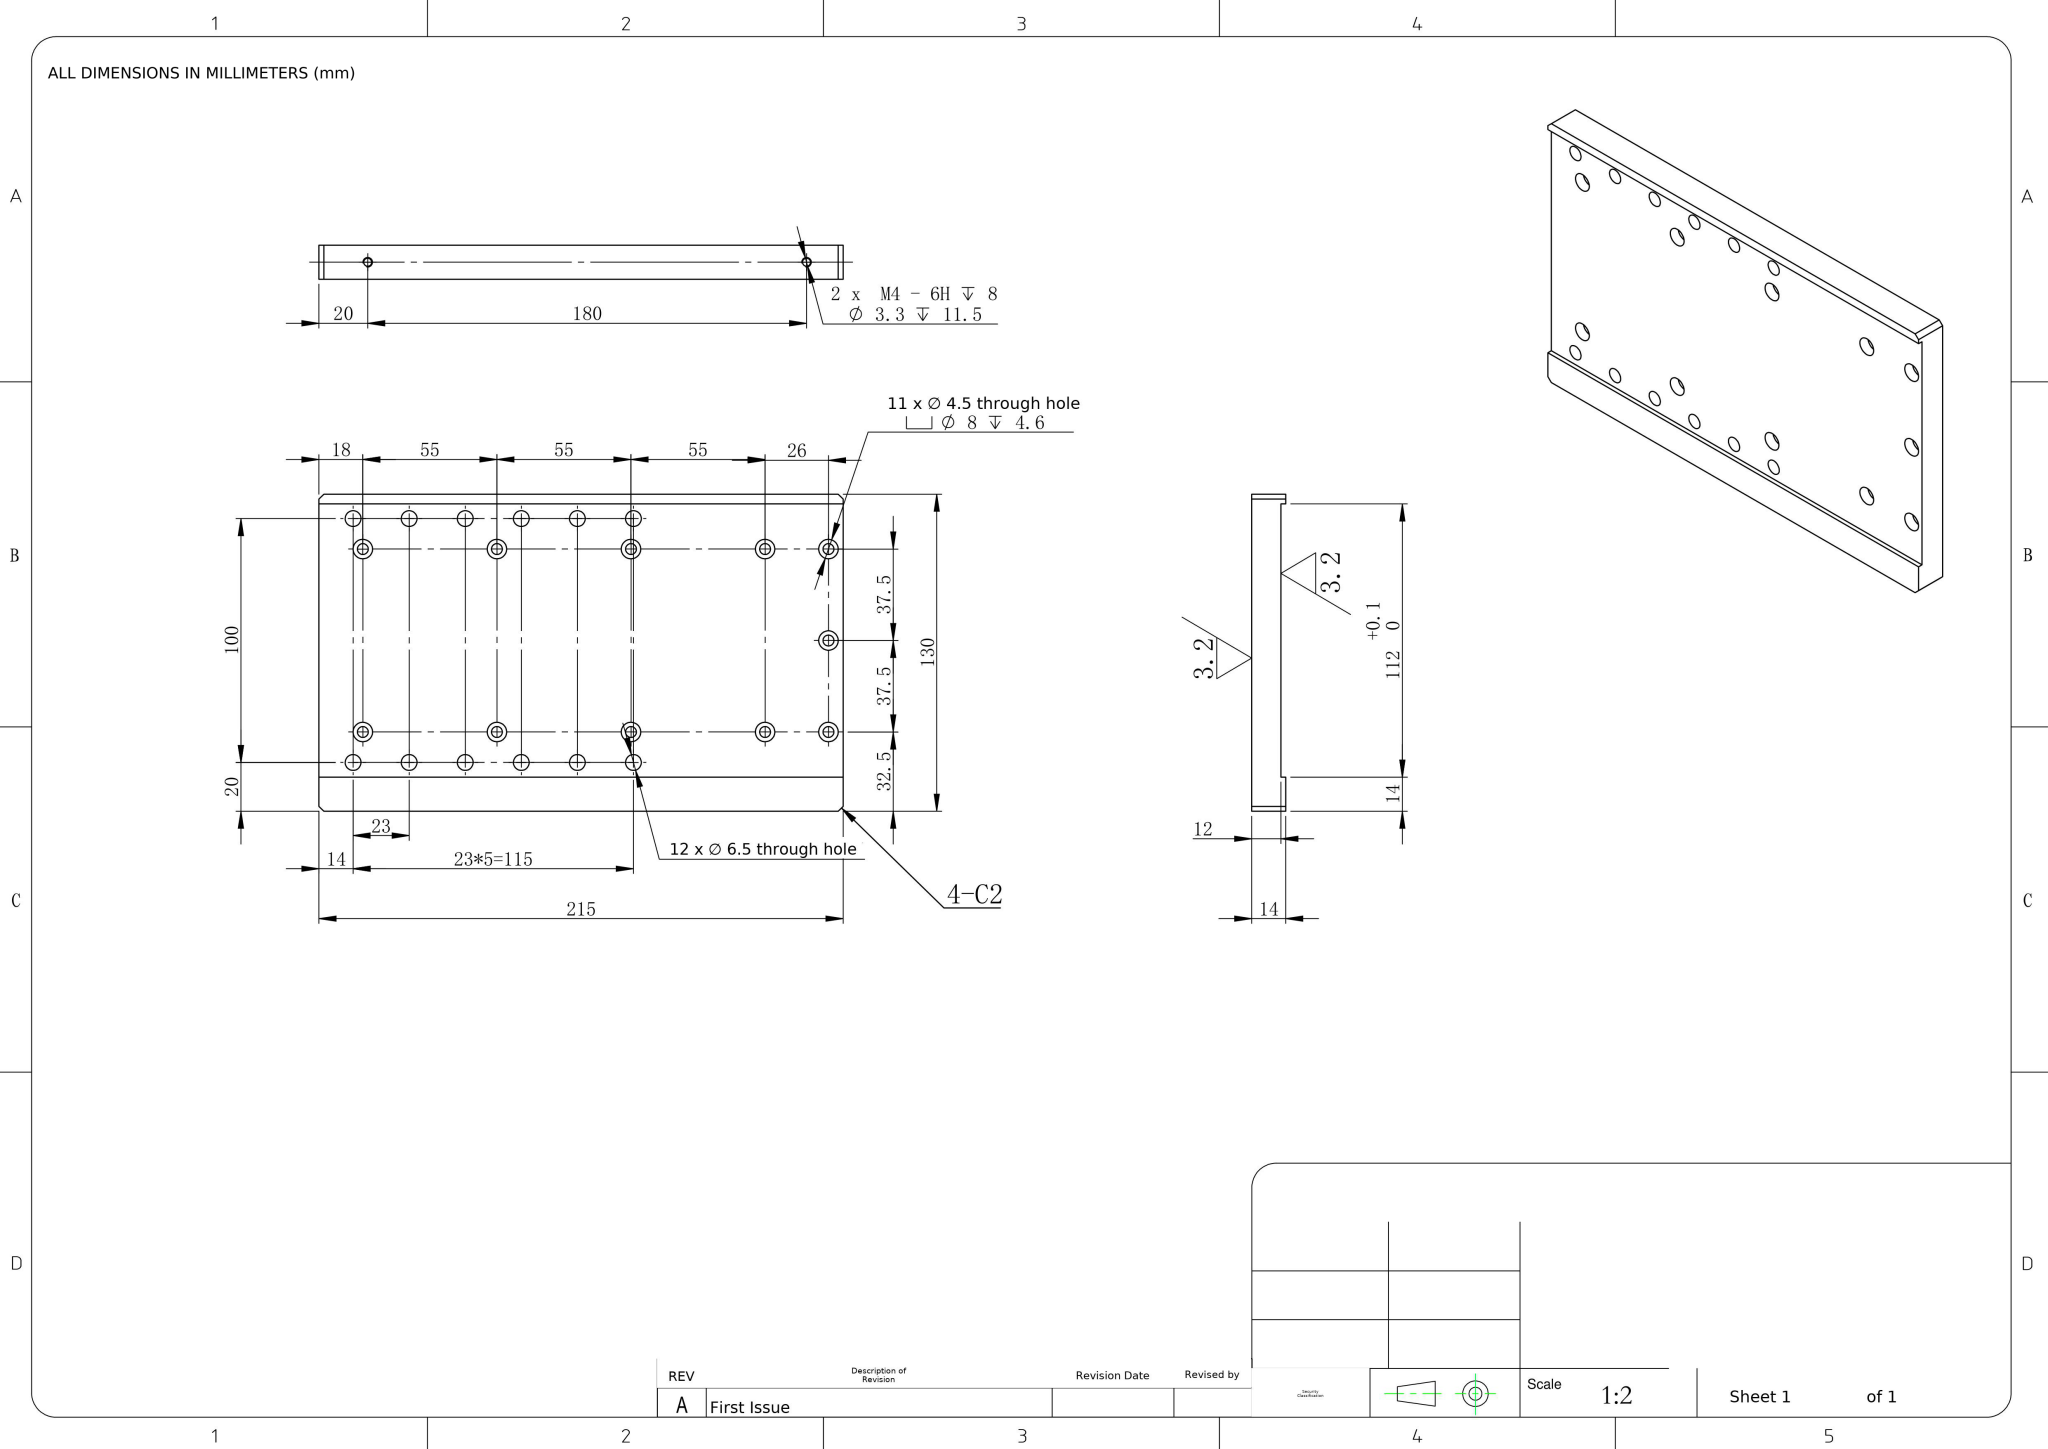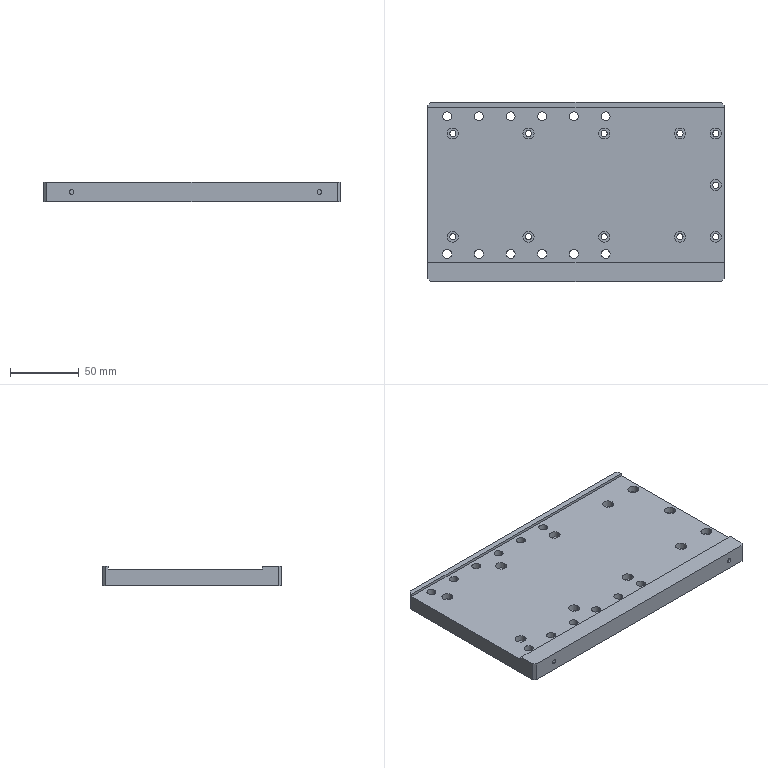Part | NX | mm | 1 solid | 99 faces | box 215 x 130 x 14 mm | volume 334215 mm3 | cylinder 72 | plane 27 | commonest cylinder face diameters 6.5 x24 8 x22 4.5 x22 3.3 x4